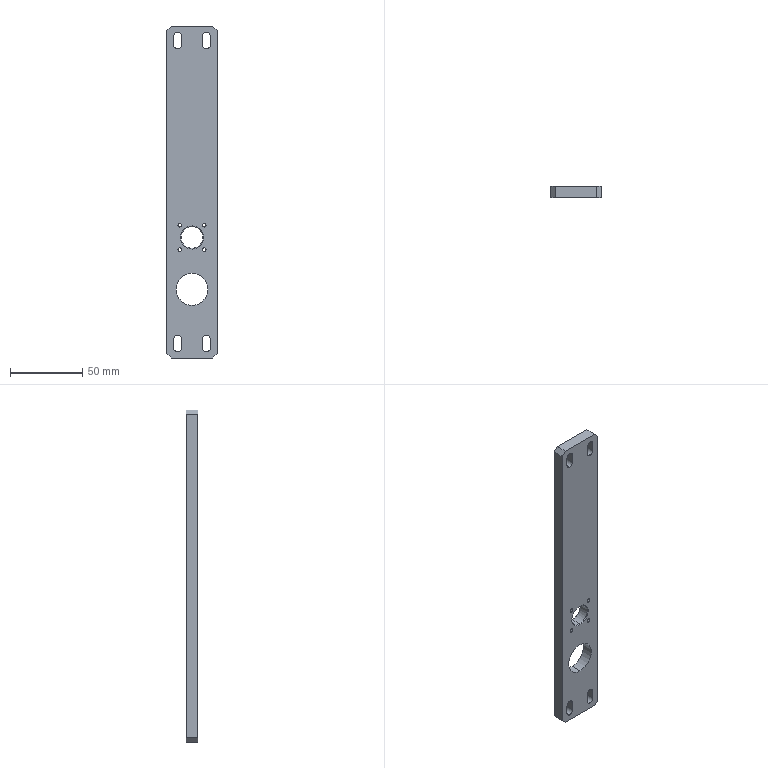Component | SolidWorks | WirePressingUnitUpperPlate-1 | 1 solid | 46 faces | box 34.8 x 7.8 x 230 mm | volume 55957 mm3 | cylinder 24 | plane 18 | cone 4 | commonest cylinder face diameters 5.5 x12 2.5 x8 22.2 x2 15 x2
build123d program:
from build123d import *

# Parameters (mm, degrees)
SKETCH1_W           = 230
SKETCH1_H           = 34.8
BOSS_EXTRUDE1_DEPTH = 3.9
CHAMFER1_SIZE       = 3
SKETCH5_R           = 7.5
CUT_EXTRUDE4_DEPTH  = 117.57
CHAMFER3_SIZE       = 0.5
M3_TAPPED_HOLE1_D   = 2.5
SKETCH10_R          = 11.1
CUT_EXTRUDE5_DEPTH  = 117.57
CUT_EXTRUDE6_DEPTH  = 117.57
LPATTERN1_COUNT     = 2
LPATTERN1_PITCH     = 210


with BuildPart() as part:
    # Sketch1 → Boss-Extrude1 (new, symmetric)
    with BuildSketch(Plane.XY):
        Rectangle(SKETCH1_W, SKETCH1_H)
    extrude(amount=BOSS_EXTRUDE1_DEPTH, both=True)

    # Chamfer1
    chamfer1_edges = [part.edges().sort_by_distance(p)[0] for p in [
        (-115, 17.4, 0),
        (115, 17.4, 0),
        (115, -17.4, 0),
        (-115, -17.4, 0),
    ]]
    chamfer(chamfer1_edges, length=CHAMFER1_SIZE)

    # Sketch5 → Cut-Extrude4 (cut, through all)
    with BuildSketch(Plane.XY.offset(3.9)):
        with Locations((31.5, 0)):
            Circle(SKETCH5_R)
    extrude(amount=-CUT_EXTRUDE4_DEPTH, mode=Mode.SUBTRACT)

    # Chamfer3
    chamfer3_edges = [part.edges().sort_by_distance(p)[0] for p in [
        (24, 0, -3.9),
        (24, 0, 3.9),
    ]]
    chamfer(chamfer3_edges, length=CHAMFER3_SIZE)

    # M3 Tapped Hole1 (through all)
    with Locations(Plane.XY.offset(3.9)):
        with Locations((23.015, 8.485), (39.985, 8.485), (39.985, -8.485), (23.015, -8.485)):
            Hole(M3_TAPPED_HOLE1_D / 2)

    # Sketch10 → Cut-Extrude5 (cut, through all)
    with BuildSketch(Plane(origin=(0, 0, -3.9), x_dir=(-1, 0, 0), z_dir=(0, 0, -1))):
        with Locations((-67.5, 0)):
            Circle(SKETCH10_R)
    extrude(amount=-CUT_EXTRUDE5_DEPTH, mode=Mode.SUBTRACT)

    # Sketch11 → Cut-Extrude6 (cut, through all)
    with BuildSketch(Plane.XY.offset(3.9)):
        with BuildLine():
            Line((-108, 12.75), (-102, 12.75))
            ThreePointArc((-102, 12.75), (-99.25, 10), (-102, 7.25))
            Line((-102, 7.25), (-108, 7.25))
            ThreePointArc((-108, 7.25), (-110.75, 10), (-108, 12.75))
        make_face()
        with BuildLine():
            Line((-108, -7.25), (-102, -7.25))
            ThreePointArc((-102, -7.25), (-99.25, -10), (-102, -12.75))
            Line((-102, -12.75), (-108, -12.75))
            ThreePointArc((-108, -12.75), (-110.75, -10), (-108, -7.25))
        make_face()
    cut_extrude6 = extrude(amount=-CUT_EXTRUDE6_DEPTH, mode=Mode.SUBTRACT)

    # LPattern1: Cut-Extrude6 ×2
    with Locations(*[(i * LPATTERN1_PITCH, 0, 0) for i in range(1, LPATTERN1_COUNT)]):
        add(cut_extrude6, mode=Mode.SUBTRACT)


solid = part.part

# Placed as in the assembly
solid = solid.moved(Location((-4.335, 68.268, -95.515), (90, 0, -90)))